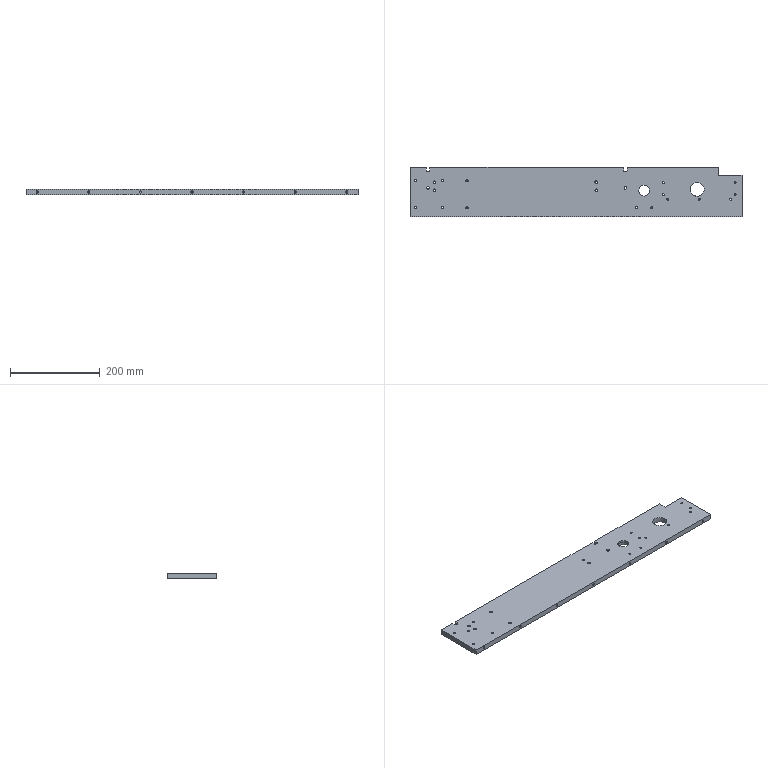Component | SolidWorks | LD101-02--Q1068-Q1-2-2 | 1 solid | 136 faces | box 740 x 110 x 12 mm | volume 937352 mm3 | cylinder 90 | plane 26 | cone 20 | commonest cylinder face diameters 5 x30 8 x14 4.5 x14 9 x8 5.5 x8 4.2 x4 6 x4 8.2 x4 | material AL6061
build123d program:
from build123d import *

# Parameters (mm, degrees)
SKETCH1_W                                          = 740
SKETCH1_H                                          = 110
BOSS_EXTRUDE1_DEPTH                                = 6
CUT_EXTRUDE1_DEPTH                                 = 375.258
M5_TAPPED_HOLE2_D                                  = 6
SKETCH9_W                                          = 52
SKETCH9_H                                          = 18
CUT_EXTRUDE2_DEPTH                                 = 375.258
SKETCH10_R                                         = 14
CUT_EXTRUDE3_DEPTH                                 = 7
SKETCH11_R                                         = 12
CUT_EXTRUDE4_DEPTH                                 = 375.131
M6_TAPPED_HOLE1_D                                  = 5
M6_TAPPED_HOLE1_DEPTH                              = 20
M6_TAPPED_HOLE1_TIP                                = 1.502
HOLE_SIZE_FOR_HEX_SOCKET_HEAD_CAP_SCRE_D           = 4.5
HOLE_SIZE_FOR_HEX_SOCKET_HEAD_CAP_SCRE_CBORE_D     = 8
HOLE_SIZE_FOR_HEX_SOCKET_HEAD_CAP_SCRE_CBORE_DEPTH = 4.6
M6_TAPPED_HOLE2_D                                  = 5
M6_TAPPED_HOLE2_DEPTH                              = 20
M6_TAPPED_HOLE2_TIP                                = 1.502
HOLE_SIZE_FOR_HEX_SOCKET_HEAD_CAP_2_D              = 5.5
HOLE_SIZE_FOR_HEX_SOCKET_HEAD_CAP_2_CBORE_D        = 9
HOLE_SIZE_FOR_HEX_SOCKET_HEAD_CAP_2_CBORE_DEPTH    = 5.7
M6_TAPPED_HOLE3_D                                  = 5
M5_TAPPED_HOLE3_D                                  = 4.2


with BuildPart() as part:
    # Sketch1 → Boss-Extrude1 (new, symmetric)
    with BuildSketch(Plane(origin=(0, 0, 0), x_dir=(1, 0, 0), z_dir=(0, 1, 0))):
        Rectangle(SKETCH1_W, SKETCH1_H)
    extrude(amount=BOSS_EXTRUDE1_DEPTH, both=True)

    # Sketch2 → Cut-Extrude1 (cut, through all)
    with BuildSketch(Plane.XZ.offset(6)):
        with BuildLine():
            Line((-325.9, 55), (-325.9, 49))
            ThreePointArc((-325.9, 49), (-330, 44.9), (-334.1, 49))
            Line((-334.1, 49), (-334.1, 55))
            ThreePointArc((-334.1, 55), (-330, 59.1), (-325.9, 55))
        make_face()
        with BuildLine():
            Line((105.9, 55), (105.9, 49))
            ThreePointArc((105.9, 49), (110, 44.9), (114.1, 49))
            Line((114.1, 49), (114.1, 55))
            ThreePointArc((114.1, 55), (110, 59.1), (105.9, 55))
        make_face()
    extrude(amount=-CUT_EXTRUDE1_DEPTH, mode=Mode.SUBTRACT)

    # M5 Tapped Hole2 (through all)
    with Locations(Plane(origin=(0, -6, 0), x_dir=(-1, 0, 0), z_dir=(0, -1, 0))):
        with Locations((330, -9), (-110, -9)):
            Hole(M5_TAPPED_HOLE2_D / 2)

    # Sketch9 → Cut-Extrude2 (cut, through all)
    with BuildSketch(Plane.XZ.offset(6)):
        with Locations((344, 46)):
            Rectangle(SKETCH9_W, SKETCH9_H)
    extrude(amount=-CUT_EXTRUDE2_DEPTH, mode=Mode.SUBTRACT)

    # Sketch10 → Cut-Extrude3 (cut)
    with BuildSketch(Plane(origin=(0, 6, 0), x_dir=(1, 0, 0), z_dir=(0, 1, 0))):
        with Locations(Location((152, -3, 0), (0, 0, 270))):
            Circle(SKETCH10_R)
    extrude(amount=-CUT_EXTRUDE3_DEPTH, mode=Mode.SUBTRACT)

    # Sketch11 → Cut-Extrude4 (cut, through all)
    with BuildSketch(Plane(origin=(0, -1, 0), x_dir=(1, 0, 0), z_dir=(0, 1, 0))):
        with Locations(Location((152, -3, 0), (0, 0, 270))):
            Circle(SKETCH11_R)
    extrude(amount=-CUT_EXTRUDE4_DEPTH, mode=Mode.SUBTRACT)

    # Sketch12 → 1 Rc Tapped Hole1 (revolve, cut)
    with BuildSketch(Plane(origin=(270, 6, 6), x_dir=(0, 0, 1), z_dir=(1, 0, 0))):
        Polygon((0, 0), (0, 38.762), (13.5, 30.65), (13.5, 19.1), (15.289, 19.1), (15.885, 0), align=None)
    revolve(axis=Axis((270, 12.35, 6), (0, -1, 0)), mode=Mode.SUBTRACT)

    # M6 Tapped Hole1
    with Locations(Plane.XY.offset(37)):
        with Locations((362, 0), (347, 0)):
            Hole(M6_TAPPED_HOLE1_D / 2, depth=M6_TAPPED_HOLE1_DEPTH)
            with Locations((0, 0, -(M6_TAPPED_HOLE1_DEPTH + M6_TAPPED_HOLE1_TIP / 2))):  # 118° drill point
                Cone(0, M6_TAPPED_HOLE1_D / 2, M6_TAPPED_HOLE1_TIP, mode=Mode.SUBTRACT)

    # Hole Size _for_ Hex Socket Head Cap Scre (through all)
    with Locations(Plane(origin=(0, 6, 0), x_dir=(1, 0, 0), z_dir=(0, 1, 0))):
        with Locations((344.5, 16), (354.5, 6), (354.5, -21), (194.5, -21), (194.5, 6), (204.5, 16), (274.5, 16)):
            CounterBoreHole(HOLE_SIZE_FOR_HEX_SOCKET_HEAD_CAP_SCRE_D / 2, HOLE_SIZE_FOR_HEX_SOCKET_HEAD_CAP_SCRE_CBORE_D / 2, HOLE_SIZE_FOR_HEX_SOCKET_HEAD_CAP_SCRE_CBORE_DEPTH)

    # M6 Tapped Hole2
    with Locations(Plane(origin=(0, 0, -55), x_dir=(-1, 0, 0), z_dir=(0, 0, -1))):
        with Locations((0, 0), (-115, 0), (-230, 0), (115, 0), (230, 0), (-345, 0), (345, 0)):
            Hole(M6_TAPPED_HOLE2_D / 2, depth=M6_TAPPED_HOLE2_DEPTH)
            with Locations((0, 0, -(M6_TAPPED_HOLE2_DEPTH + M6_TAPPED_HOLE2_TIP / 2))):  # 118° drill point
                Cone(0, M6_TAPPED_HOLE2_D / 2, M6_TAPPED_HOLE2_TIP, mode=Mode.SUBTRACT)

    # Hole Size _for_ Hex Socket Head Cap  2 (through all)
    with Locations(Plane(origin=(0, 6, 0), x_dir=(1, 0, 0), z_dir=(0, 1, 0))):
        with Locations((45, -22), (45, -4), (-315, -22), (-315, -4)):
            CounterBoreHole(HOLE_SIZE_FOR_HEX_SOCKET_HEAD_CAP_2_D / 2, HOLE_SIZE_FOR_HEX_SOCKET_HEAD_CAP_2_CBORE_D / 2, HOLE_SIZE_FOR_HEX_SOCKET_HEAD_CAP_2_CBORE_DEPTH)

    # M6 Tapped Hole3 (through all)
    with Locations(Plane(origin=(0, 6, 0), x_dir=(1, 0, 0), z_dir=(0, 1, 0))):
        with Locations((-243, -25), (-243, 35), (-298, -25), (-298, 35), (-358, -25), (-358, 35)):
            Hole(M6_TAPPED_HOLE3_D / 2)

    # M5 Tapped Hole3 (through all)
    with Locations(Plane(origin=(0, 6, 0), x_dir=(1, 0, 0), z_dir=(0, 1, 0))):
        with Locations((169, 35), (135, 35)):
            Hole(M5_TAPPED_HOLE3_D / 2)


solid = part.part

# Placed as in the assembly
solid = solid.moved(Location((-30.29, -184.897, 5.257), (-90, 0, 0)))